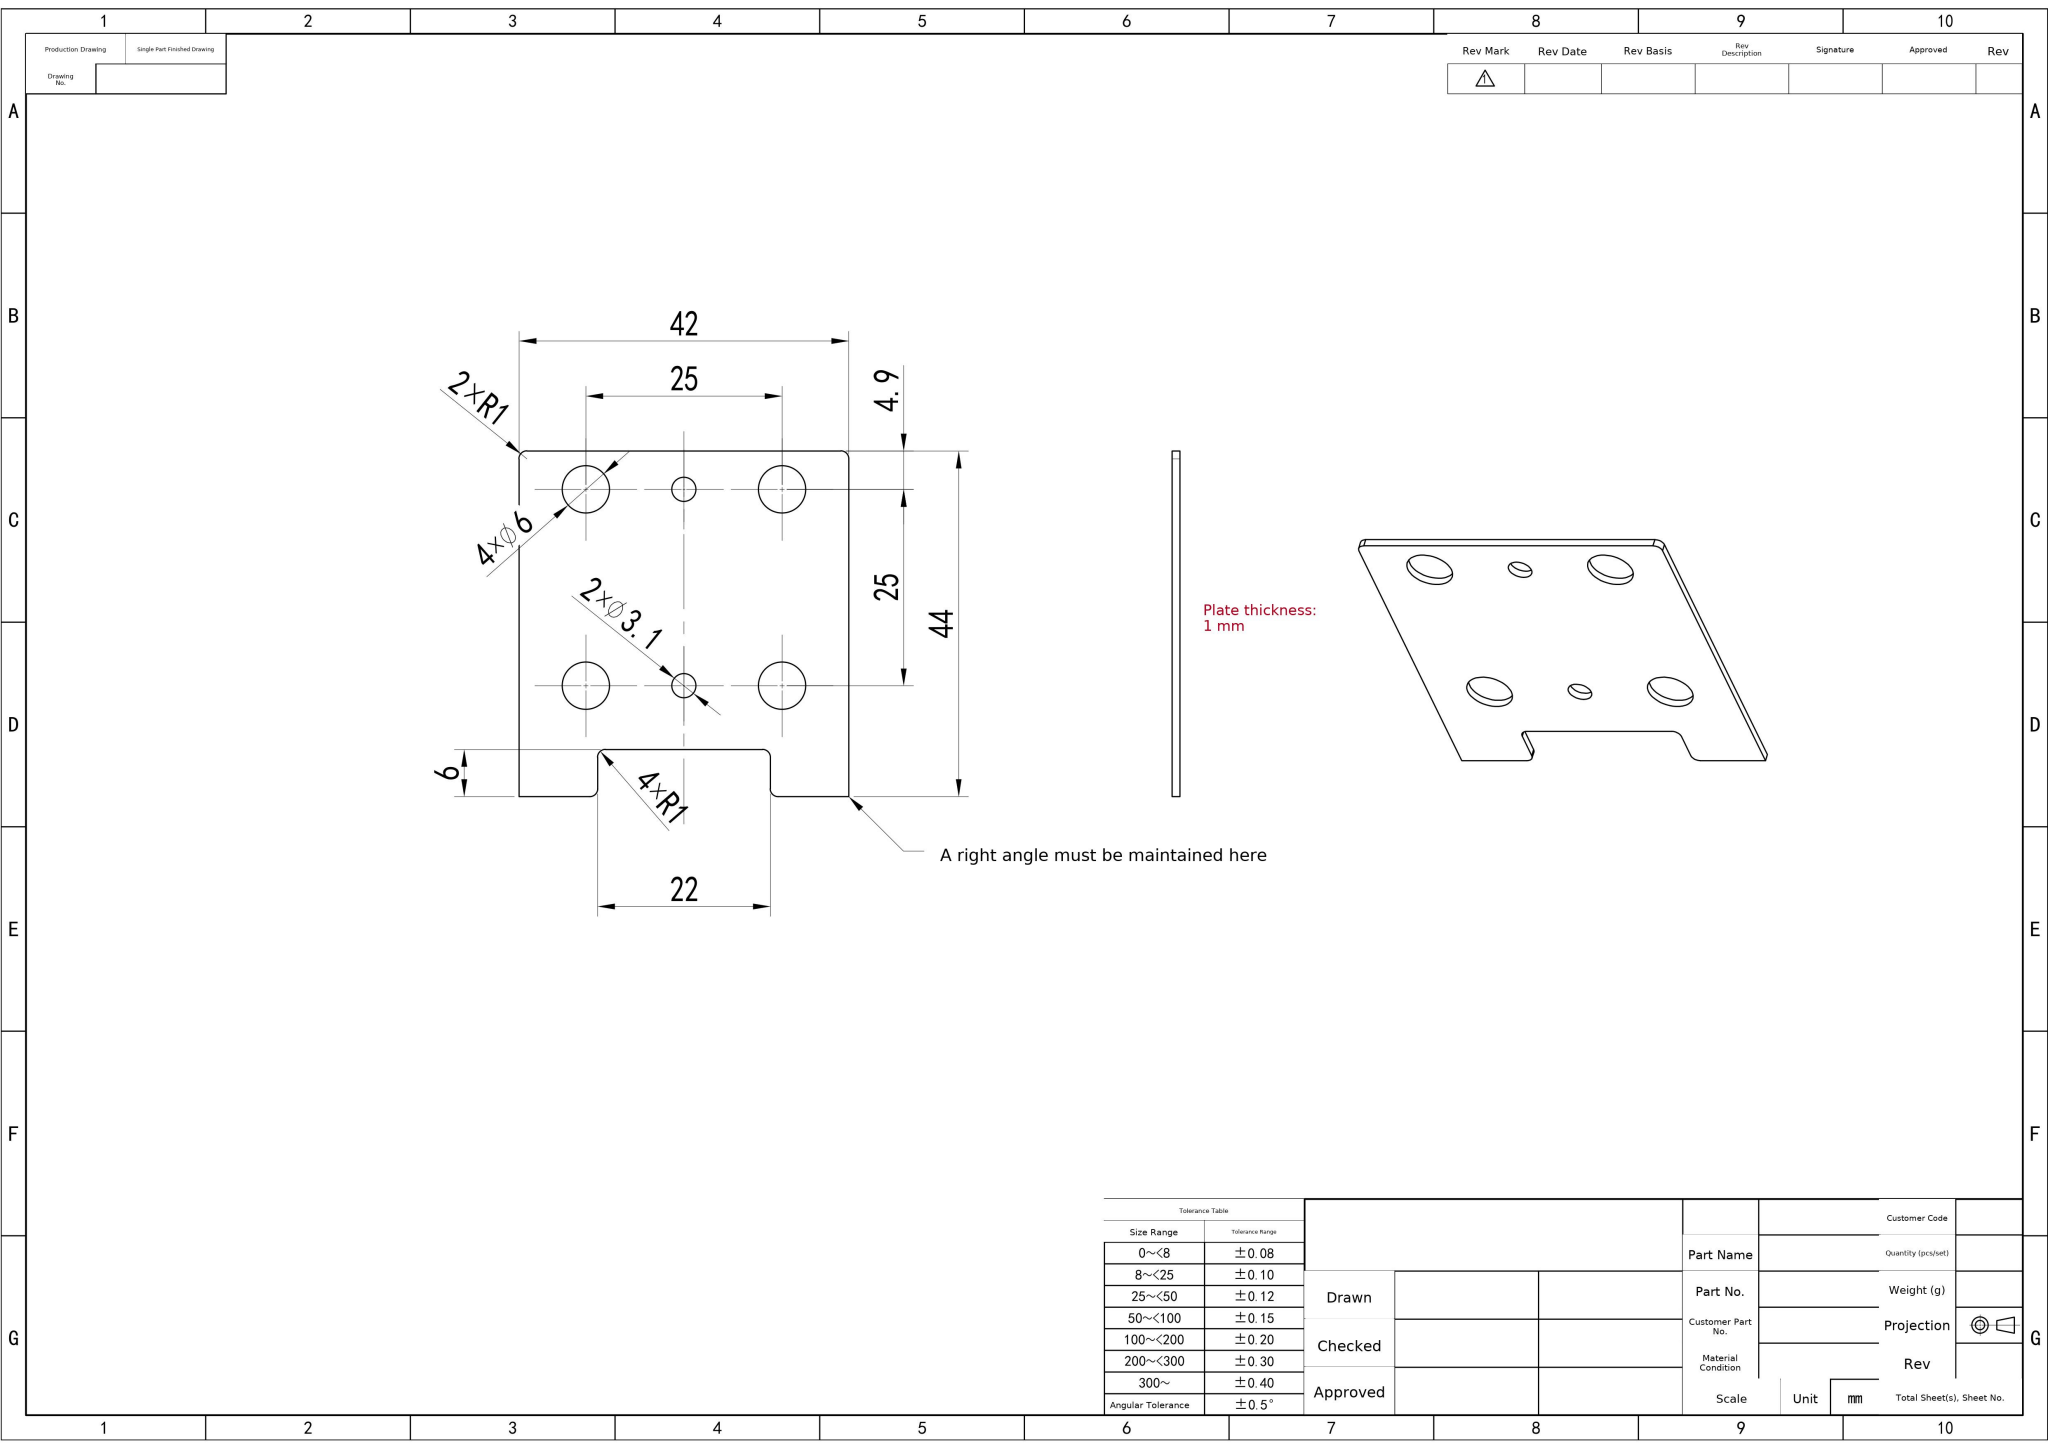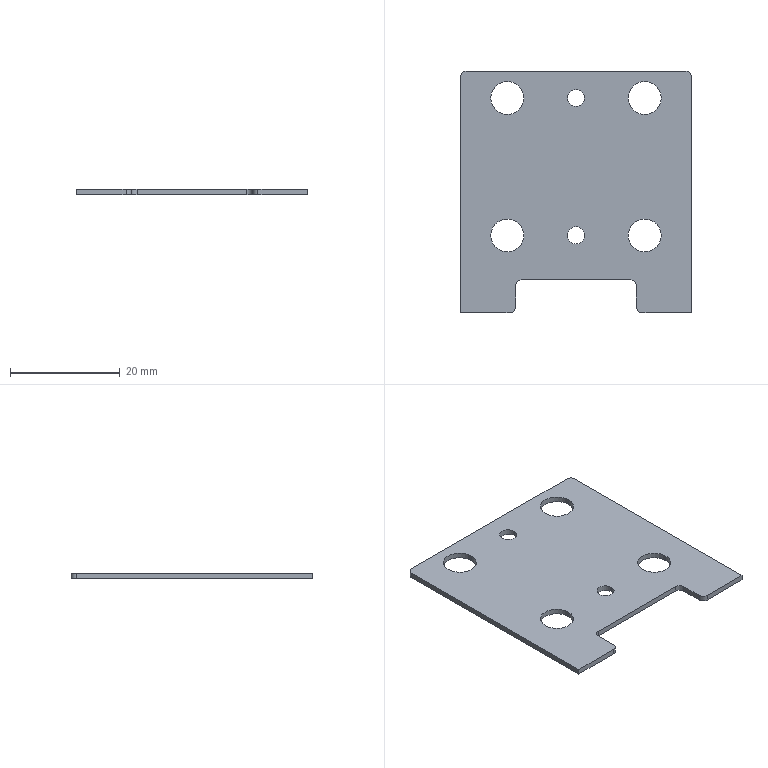Part | SolidWorks | mm | 1 solid | 28 faces | box 42 x 44 x 1 mm | volume 1587 mm3 | cylinder 18 | plane 10 | commonest cylinder face diameters 6 x8 2 x6 3.1 x4
STEP:
#1=CARTESIAN_POINT('',(15.5,0.,1.));
#2=VERTEX_POINT('',#1);
#3=CARTESIAN_POINT('',(9.5,0.,1.));
#4=VERTEX_POINT('',#3);
#5=CARTESIAN_POINT('',(12.5,0.,1.));
#6=DIRECTION('',(0.,0.,-1.));
#7=DIRECTION('',(-1.,0.,0.));
#8=AXIS2_PLACEMENT_3D('',#5,#6,#7);
#9=CIRCLE('',#8,3.);
#10=EDGE_CURVE('',#2,#4,#9,.T.);
#11=ORIENTED_EDGE('',*,*,#10,.F.);
#12=CARTESIAN_POINT('',(15.5,0.,0.));
#13=VERTEX_POINT('',#12);
#14=CARTESIAN_POINT('',(15.5,0.,1.));
#15=DIRECTION('',(0.,0.,-1.));
#16=VECTOR('',#15,1000.);
#17=LINE('',#14,#16);
#18=EDGE_CURVE('',#2,#13,#17,.T.);
#19=ORIENTED_EDGE('',*,*,#18,.T.);
#20=CARTESIAN_POINT('',(9.5,0.,0.));
#21=VERTEX_POINT('',#20);
#22=CARTESIAN_POINT('',(12.5,0.,0.));
#23=DIRECTION('',(0.,0.,1.));
#24=DIRECTION('',(-1.,0.,0.));
#25=AXIS2_PLACEMENT_3D('',#22,#23,#24);
#26=CIRCLE('',#25,3.);
#27=EDGE_CURVE('',#21,#13,#26,.T.);
#28=ORIENTED_EDGE('',*,*,#27,.F.);
#29=CARTESIAN_POINT('',(9.5,0.,1.));
#30=DIRECTION('',(0.,0.,-1.));
#31=VECTOR('',#30,1000.);
#32=LINE('',#29,#31);
#33=EDGE_CURVE('',#4,#21,#32,.T.);
#34=ORIENTED_EDGE('',*,*,#33,.F.);
#35=EDGE_LOOP('',(#11,#19,#28,#34));
#36=FACE_OUTER_BOUND('',#35,.T.);
#37=CARTESIAN_POINT('',(12.5,0.,1.));
#38=DIRECTION('',(0.,0.,-1.));
#39=DIRECTION('',(-1.,0.,0.));
#40=AXIS2_PLACEMENT_3D('',#37,#38,#39);
#41=CYLINDRICAL_SURFACE('',#40,3.);
#42=ADVANCED_FACE('',(#36),#41,.F.);
#43=CARTESIAN_POINT('',(15.5,-25.,1.));
#44=VERTEX_POINT('',#43);
#45=CARTESIAN_POINT('',(9.5,-25.,1.));
#46=VERTEX_POINT('',#45);
#47=CARTESIAN_POINT('',(12.5,-25.,1.));
#48=DIRECTION('',(0.,0.,-1.));
#49=DIRECTION('',(-1.,0.,0.));
#50=AXIS2_PLACEMENT_3D('',#47,#48,#49);
#51=CIRCLE('',#50,3.);
#52=EDGE_CURVE('',#44,#46,#51,.T.);
#53=ORIENTED_EDGE('',*,*,#52,.F.);
#54=CARTESIAN_POINT('',(15.5,-25.,0.));
#55=VERTEX_POINT('',#54);
#56=CARTESIAN_POINT('',(15.5,-25.,1.));
#57=DIRECTION('',(0.,0.,-1.));
#58=VECTOR('',#57,1000.);
#59=LINE('',#56,#58);
#60=EDGE_CURVE('',#44,#55,#59,.T.);
#61=ORIENTED_EDGE('',*,*,#60,.T.);
#62=CARTESIAN_POINT('',(9.5,-25.,0.));
#63=VERTEX_POINT('',#62);
#64=CARTESIAN_POINT('',(12.5,-25.,0.));
#65=DIRECTION('',(0.,0.,1.));
#66=DIRECTION('',(-1.,0.,0.));
#67=AXIS2_PLACEMENT_3D('',#64,#65,#66);
#68=CIRCLE('',#67,3.);
#69=EDGE_CURVE('',#63,#55,#68,.T.);
#70=ORIENTED_EDGE('',*,*,#69,.F.);
#71=CARTESIAN_POINT('',(9.5,-25.,1.));
#72=DIRECTION('',(0.,0.,-1.));
#73=VECTOR('',#72,1000.);
#74=LINE('',#71,#73);
#75=EDGE_CURVE('',#46,#63,#74,.T.);
#76=ORIENTED_EDGE('',*,*,#75,.F.);
#77=EDGE_LOOP('',(#53,#61,#70,#76));
#78=FACE_OUTER_BOUND('',#77,.T.);
#79=CARTESIAN_POINT('',(12.5,-25.,1.));
#80=DIRECTION('',(0.,0.,-1.));
#81=DIRECTION('',(-1.,0.,0.));
#82=AXIS2_PLACEMENT_3D('',#79,#80,#81);
#83=CYLINDRICAL_SURFACE('',#82,3.);
#84=ADVANCED_FACE('',(#78),#83,.F.);
#85=CARTESIAN_POINT('',(1.55,0.,1.));
#86=VERTEX_POINT('',#85);
#87=CARTESIAN_POINT('',(-1.55,0.,1.));
#88=VERTEX_POINT('',#87);
#89=CARTESIAN_POINT('',(0.,0.,1.));
#90=DIRECTION('',(0.,0.,-1.));
#91=DIRECTION('',(-1.,0.,0.));
#92=AXIS2_PLACEMENT_3D('',#89,#90,#91);
#93=CIRCLE('',#92,1.55);
#94=EDGE_CURVE('',#86,#88,#93,.T.);
#95=ORIENTED_EDGE('',*,*,#94,.F.);
#96=CARTESIAN_POINT('',(1.55,0.,0.));
#97=VERTEX_POINT('',#96);
#98=CARTESIAN_POINT('',(1.55,0.,1.));
#99=DIRECTION('',(0.,0.,-1.));
#100=VECTOR('',#99,1000.);
#101=LINE('',#98,#100);
#102=EDGE_CURVE('',#86,#97,#101,.T.);
#103=ORIENTED_EDGE('',*,*,#102,.T.);
#104=CARTESIAN_POINT('',(-1.55,0.,0.));
#105=VERTEX_POINT('',#104);
#106=CARTESIAN_POINT('',(0.,0.,0.));
#107=DIRECTION('',(0.,0.,1.));
#108=DIRECTION('',(-1.,0.,0.));
#109=AXIS2_PLACEMENT_3D('',#106,#107,#108);
#110=CIRCLE('',#109,1.55);
#111=EDGE_CURVE('',#105,#97,#110,.T.);
#112=ORIENTED_EDGE('',*,*,#111,.F.);
#113=CARTESIAN_POINT('',(-1.55,0.,1.));
#114=DIRECTION('',(0.,0.,-1.));
#115=VECTOR('',#114,1000.);
#116=LINE('',#113,#115);
#117=EDGE_CURVE('',#88,#105,#116,.T.);
#118=ORIENTED_EDGE('',*,*,#117,.F.);
#119=EDGE_LOOP('',(#95,#103,#112,#118));
#120=FACE_OUTER_BOUND('',#119,.T.);
#121=CARTESIAN_POINT('',(0.,0.,1.));
#122=DIRECTION('',(0.,0.,-1.));
#123=DIRECTION('',(-1.,0.,0.));
#124=AXIS2_PLACEMENT_3D('',#121,#122,#123);
#125=CYLINDRICAL_SURFACE('',#124,1.55);
#126=ADVANCED_FACE('',(#120),#125,.F.);
#127=CARTESIAN_POINT('',(1.55,-25.,1.));
#128=VERTEX_POINT('',#127);
#129=CARTESIAN_POINT('',(-1.55,-25.,1.));
#130=VERTEX_POINT('',#129);
#131=CARTESIAN_POINT('',(0.,-25.,1.));
#132=DIRECTION('',(0.,0.,-1.));
#133=DIRECTION('',(-1.,0.,0.));
#134=AXIS2_PLACEMENT_3D('',#131,#132,#133);
#135=CIRCLE('',#134,1.55);
#136=EDGE_CURVE('',#128,#130,#135,.T.);
#137=ORIENTED_EDGE('',*,*,#136,.F.);
#138=CARTESIAN_POINT('',(1.55,-25.,0.));
#139=VERTEX_POINT('',#138);
#140=CARTESIAN_POINT('',(1.55,-25.,1.));
#141=DIRECTION('',(0.,0.,-1.));
#142=VECTOR('',#141,1000.);
#143=LINE('',#140,#142);
#144=EDGE_CURVE('',#128,#139,#143,.T.);
#145=ORIENTED_EDGE('',*,*,#144,.T.);
#146=CARTESIAN_POINT('',(-1.55,-25.,0.));
#147=VERTEX_POINT('',#146);
#148=CARTESIAN_POINT('',(0.,-25.,0.));
#149=DIRECTION('',(0.,0.,1.));
#150=DIRECTION('',(-1.,0.,0.));
#151=AXIS2_PLACEMENT_3D('',#148,#149,#150);
#152=CIRCLE('',#151,1.55);
#153=EDGE_CURVE('',#147,#139,#152,.T.);
#154=ORIENTED_EDGE('',*,*,#153,.F.);
#155=CARTESIAN_POINT('',(-1.55,-25.,1.));
#156=DIRECTION('',(0.,0.,-1.));
#157=VECTOR('',#156,1000.);
#158=LINE('',#155,#157);
#159=EDGE_CURVE('',#130,#147,#158,.T.);
#160=ORIENTED_EDGE('',*,*,#159,.F.);
#161=EDGE_LOOP('',(#137,#145,#154,#160));
#162=FACE_OUTER_BOUND('',#161,.T.);
#163=CARTESIAN_POINT('',(0.,-25.,1.));
#164=DIRECTION('',(0.,0.,-1.));
#165=DIRECTION('',(-1.,0.,0.));
#166=AXIS2_PLACEMENT_3D('',#163,#164,#165);
#167=CYLINDRICAL_SURFACE('',#166,1.55);
#168=ADVANCED_FACE('',(#162),#167,.F.);
#169=CARTESIAN_POINT('',(-9.5,0.,1.));
#170=VERTEX_POINT('',#169);
#171=CARTESIAN_POINT('',(-15.5,0.,1.));
#172=VERTEX_POINT('',#171);
#173=CARTESIAN_POINT('',(-12.5,0.,1.));
#174=DIRECTION('',(0.,0.,-1.));
#175=DIRECTION('',(-1.,0.,0.));
#176=AXIS2_PLACEMENT_3D('',#173,#174,#175);
#177=CIRCLE('',#176,3.);
#178=EDGE_CURVE('',#170,#172,#177,.T.);
#179=ORIENTED_EDGE('',*,*,#178,.F.);
#180=CARTESIAN_POINT('',(-9.5,0.,0.));
#181=VERTEX_POINT('',#180);
#182=CARTESIAN_POINT('',(-9.5,0.,1.));
#183=DIRECTION('',(0.,0.,-1.));
#184=VECTOR('',#183,1000.);
#185=LINE('',#182,#184);
#186=EDGE_CURVE('',#170,#181,#185,.T.);
#187=ORIENTED_EDGE('',*,*,#186,.T.);
#188=CARTESIAN_POINT('',(-15.5,0.,0.));
#189=VERTEX_POINT('',#188);
#190=CARTESIAN_POINT('',(-12.5,0.,0.));
#191=DIRECTION('',(0.,0.,1.));
#192=DIRECTION('',(-1.,0.,0.));
#193=AXIS2_PLACEMENT_3D('',#190,#191,#192);
#194=CIRCLE('',#193,3.);
#195=EDGE_CURVE('',#189,#181,#194,.T.);
#196=ORIENTED_EDGE('',*,*,#195,.F.);
#197=CARTESIAN_POINT('',(-15.5,0.,1.));
#198=DIRECTION('',(0.,0.,-1.));
#199=VECTOR('',#198,1000.);
#200=LINE('',#197,#199);
#201=EDGE_CURVE('',#172,#189,#200,.T.);
#202=ORIENTED_EDGE('',*,*,#201,.F.);
#203=EDGE_LOOP('',(#179,#187,#196,#202));
#204=FACE_OUTER_BOUND('',#203,.T.);
#205=CARTESIAN_POINT('',(-12.5,0.,1.));
#206=DIRECTION('',(0.,0.,-1.));
#207=DIRECTION('',(-1.,0.,0.));
#208=AXIS2_PLACEMENT_3D('',#205,#206,#207);
#209=CYLINDRICAL_SURFACE('',#208,3.);
#210=ADVANCED_FACE('',(#204),#209,.F.);
#211=CARTESIAN_POINT('',(-9.5,-25.,1.));
#212=VERTEX_POINT('',#211);
#213=CARTESIAN_POINT('',(-15.5,-25.,1.));
#214=VERTEX_POINT('',#213);
#215=CARTESIAN_POINT('',(-12.5,-25.,1.));
#216=DIRECTION('',(0.,0.,-1.));
#217=DIRECTION('',(-1.,0.,0.));
#218=AXIS2_PLACEMENT_3D('',#215,#216,#217);
#219=CIRCLE('',#218,3.);
#220=EDGE_CURVE('',#212,#214,#219,.T.);
#221=ORIENTED_EDGE('',*,*,#220,.F.);
#222=CARTESIAN_POINT('',(-9.5,-25.,0.));
#223=VERTEX_POINT('',#222);
#224=CARTESIAN_POINT('',(-9.5,-25.,1.));
#225=DIRECTION('',(0.,0.,-1.));
#226=VECTOR('',#225,1000.);
#227=LINE('',#224,#226);
#228=EDGE_CURVE('',#212,#223,#227,.T.);
#229=ORIENTED_EDGE('',*,*,#228,.T.);
#230=CARTESIAN_POINT('',(-15.5,-25.,0.));
#231=VERTEX_POINT('',#230);
#232=CARTESIAN_POINT('',(-12.5,-25.,0.));
#233=DIRECTION('',(0.,0.,1.));
#234=DIRECTION('',(-1.,0.,0.));
#235=AXIS2_PLACEMENT_3D('',#232,#233,#234);
#236=CIRCLE('',#235,3.);
#237=EDGE_CURVE('',#231,#223,#236,.T.);
#238=ORIENTED_EDGE('',*,*,#237,.F.);
#239=CARTESIAN_POINT('',(-15.5,-25.,1.));
#240=DIRECTION('',(0.,0.,-1.));
#241=VECTOR('',#240,1000.);
#242=LINE('',#239,#241);
#243=EDGE_CURVE('',#214,#231,#242,.T.);
#244=ORIENTED_EDGE('',*,*,#243,.F.);
#245=EDGE_LOOP('',(#221,#229,#238,#244));
#246=FACE_OUTER_BOUND('',#245,.T.);
#247=CARTESIAN_POINT('',(-12.5,-25.,1.));
#248=DIRECTION('',(0.,0.,-1.));
#249=DIRECTION('',(-1.,0.,0.));
#250=AXIS2_PLACEMENT_3D('',#247,#248,#249);
#251=CYLINDRICAL_SURFACE('',#250,3.);
#252=ADVANCED_FACE('',(#246),#251,.F.);
#253=CARTESIAN_POINT('',(12.5,0.,1.));
#254=DIRECTION('',(0.,0.,-1.));
#255=DIRECTION('',(-1.,0.,0.));
#256=AXIS2_PLACEMENT_3D('',#253,#254,#255);
#257=CIRCLE('',#256,3.);
#258=EDGE_CURVE('',#4,#2,#257,.T.);
#259=ORIENTED_EDGE('',*,*,#258,.T.);
#260=ORIENTED_EDGE('',*,*,#10,.T.);
#261=EDGE_LOOP('',(#259,#260));
#262=FACE_BOUND('',#261,.T.);
#263=CARTESIAN_POINT('',(12.5,-25.,1.));
#264=DIRECTION('',(0.,0.,-1.));
#265=DIRECTION('',(-1.,0.,0.));
#266=AXIS2_PLACEMENT_3D('',#263,#264,#265);
#267=CIRCLE('',#266,3.);
#268=EDGE_CURVE('',#46,#44,#267,.T.);
#269=ORIENTED_EDGE('',*,*,#268,.T.);
#270=ORIENTED_EDGE('',*,*,#52,.T.);
#271=EDGE_LOOP('',(#269,#270));
#272=FACE_BOUND('',#271,.T.);
#273=CARTESIAN_POINT('',(0.,0.,1.));
#274=DIRECTION('',(0.,0.,-1.));
#275=DIRECTION('',(-1.,0.,0.));
#276=AXIS2_PLACEMENT_3D('',#273,#274,#275);
#277=CIRCLE('',#276,1.55);
#278=EDGE_CURVE('',#88,#86,#277,.T.);
#279=ORIENTED_EDGE('',*,*,#278,.T.);
#280=ORIENTED_EDGE('',*,*,#94,.T.);
#281=EDGE_LOOP('',(#279,#280));
#282=FACE_BOUND('',#281,.T.);
#283=CARTESIAN_POINT('',(0.,-25.,1.));
#284=DIRECTION('',(0.,0.,-1.));
#285=DIRECTION('',(-1.,0.,0.));
#286=AXIS2_PLACEMENT_3D('',#283,#284,#285);
#287=CIRCLE('',#286,1.55);
#288=EDGE_CURVE('',#130,#128,#287,.T.);
#289=ORIENTED_EDGE('',*,*,#288,.T.);
#290=ORIENTED_EDGE('',*,*,#136,.T.);
#291=EDGE_LOOP('',(#289,#290));
#292=FACE_BOUND('',#291,.T.);
#293=CARTESIAN_POINT('',(-12.5,0.,1.));
#294=DIRECTION('',(0.,0.,-1.));
#295=DIRECTION('',(-1.,0.,0.));
#296=AXIS2_PLACEMENT_3D('',#293,#294,#295);
#297=CIRCLE('',#296,3.);
#298=EDGE_CURVE('',#172,#170,#297,.T.);
#299=ORIENTED_EDGE('',*,*,#298,.T.);
#300=ORIENTED_EDGE('',*,*,#178,.T.);
#301=EDGE_LOOP('',(#299,#300));
#302=FACE_BOUND('',#301,.T.);
#303=CARTESIAN_POINT('',(-12.5,-25.,1.));
#304=DIRECTION('',(0.,0.,-1.));
#305=DIRECTION('',(-1.,0.,0.));
#306=AXIS2_PLACEMENT_3D('',#303,#304,#305);
#307=CIRCLE('',#306,3.);
#308=EDGE_CURVE('',#214,#212,#307,.T.);
#309=ORIENTED_EDGE('',*,*,#308,.T.);
#310=ORIENTED_EDGE('',*,*,#220,.T.);
#311=EDGE_LOOP('',(#309,#310));
#312=FACE_BOUND('',#311,.T.);
#313=CARTESIAN_POINT('',(20.,4.9,1.));
#314=VERTEX_POINT('',#313);
#315=CARTESIAN_POINT('',(-20.,4.9,1.));
#316=VERTEX_POINT('',#315);
#317=CARTESIAN_POINT('',(-12.,4.9,1.));
#318=DIRECTION('',(-1.,0.,0.));
#319=VECTOR('',#318,1000.);
#320=LINE('',#317,#319);
#321=EDGE_CURVE('',#314,#316,#320,.T.);
#322=ORIENTED_EDGE('',*,*,#321,.T.);
#323=CARTESIAN_POINT('',(-21.,3.9,1.));
#324=VERTEX_POINT('',#323);
#325=CARTESIAN_POINT('',(-20.,3.9,1.));
#326=DIRECTION('',(0.,0.,1.));
#327=DIRECTION('',(-1.,0.,0.));
#328=AXIS2_PLACEMENT_3D('',#325,#326,#327);
#329=CIRCLE('',#328,1.);
#330=EDGE_CURVE('',#316,#324,#329,.T.);
#331=ORIENTED_EDGE('',*,*,#330,.T.);
#332=CARTESIAN_POINT('',(-21.,-39.1,1.));
#333=VERTEX_POINT('',#332);
#334=CARTESIAN_POINT('',(-21.,-38.1,1.));
#335=DIRECTION('',(0.,-1.,0.));
#336=VECTOR('',#335,1000.);
#337=LINE('',#334,#336);
#338=EDGE_CURVE('',#324,#333,#337,.T.);
#339=ORIENTED_EDGE('',*,*,#338,.T.);
#340=CARTESIAN_POINT('',(-12.,-39.1,1.));
#341=VERTEX_POINT('',#340);
#342=CARTESIAN_POINT('',(-12.,-39.1,1.));
#343=DIRECTION('',(1.,0.,0.));
#344=VECTOR('',#343,1000.);
#345=LINE('',#342,#344);
#346=EDGE_CURVE('',#333,#341,#345,.T.);
#347=ORIENTED_EDGE('',*,*,#346,.T.);
#348=CARTESIAN_POINT('',(-11.,-38.1,1.));
#349=VERTEX_POINT('',#348);
#350=CARTESIAN_POINT('',(-12.,-38.1,1.));
#351=DIRECTION('',(0.,0.,1.));
#352=DIRECTION('',(-1.,0.,0.));
#353=AXIS2_PLACEMENT_3D('',#350,#351,#352);
#354=CIRCLE('',#353,1.);
#355=EDGE_CURVE('',#341,#349,#354,.T.);
#356=ORIENTED_EDGE('',*,*,#355,.T.);
#357=CARTESIAN_POINT('',(-11.,-34.1,1.));
#358=VERTEX_POINT('',#357);
#359=CARTESIAN_POINT('',(-11.,-38.1,1.));
#360=DIRECTION('',(0.,1.,0.));
#361=VECTOR('',#360,1000.);
#362=LINE('',#359,#361);
#363=EDGE_CURVE('',#349,#358,#362,.T.);
#364=ORIENTED_EDGE('',*,*,#363,.T.);
#365=CARTESIAN_POINT('',(-10.,-33.1,1.));
#366=VERTEX_POINT('',#365);
#367=CARTESIAN_POINT('',(-10.,-34.1,1.));
#368=DIRECTION('',(0.,0.,-1.));
#369=DIRECTION('',(-1.,0.,0.));
#370=AXIS2_PLACEMENT_3D('',#367,#368,#369);
#371=CIRCLE('',#370,1.);
#372=EDGE_CURVE('',#358,#366,#371,.T.);
#373=ORIENTED_EDGE('',*,*,#372,.T.);
#374=CARTESIAN_POINT('',(10.,-33.1,1.));
#375=VERTEX_POINT('',#374);
#376=CARTESIAN_POINT('',(-12.,-33.1,1.));
#377=DIRECTION('',(1.,0.,0.));
#378=VECTOR('',#377,1000.);
#379=LINE('',#376,#378);
#380=EDGE_CURVE('',#366,#375,#379,.T.);
#381=ORIENTED_EDGE('',*,*,#380,.T.);
#382=CARTESIAN_POINT('',(11.,-34.1,1.));
#383=VERTEX_POINT('',#382);
#384=CARTESIAN_POINT('',(10.,-34.1,1.));
#385=DIRECTION('',(0.,0.,-1.));
#386=DIRECTION('',(-1.,0.,0.));
#387=AXIS2_PLACEMENT_3D('',#384,#385,#386);
#388=CIRCLE('',#387,1.);
#389=EDGE_CURVE('',#375,#383,#388,.T.);
#390=ORIENTED_EDGE('',*,*,#389,.T.);
#391=CARTESIAN_POINT('',(11.,-38.1,1.));
#392=VERTEX_POINT('',#391);
#393=CARTESIAN_POINT('',(11.,-38.1,1.));
#394=DIRECTION('',(0.,-1.,0.));
#395=VECTOR('',#394,1000.);
#396=LINE('',#393,#395);
#397=EDGE_CURVE('',#383,#392,#396,.T.);
#398=ORIENTED_EDGE('',*,*,#397,.T.);
#399=CARTESIAN_POINT('',(12.,-39.1,1.));
#400=VERTEX_POINT('',#399);
#401=CARTESIAN_POINT('',(12.,-38.1,1.));
#402=DIRECTION('',(0.,0.,1.));
#403=DIRECTION('',(-1.,0.,0.));
#404=AXIS2_PLACEMENT_3D('',#401,#402,#403);
#405=CIRCLE('',#404,1.);
#406=EDGE_CURVE('',#392,#400,#405,.T.);
#407=ORIENTED_EDGE('',*,*,#406,.T.);
#408=CARTESIAN_POINT('',(21.,-39.1,1.));
#409=VERTEX_POINT('',#408);
#410=CARTESIAN_POINT('',(-12.,-39.1,1.));
#411=DIRECTION('',(1.,0.,0.));
#412=VECTOR('',#411,1000.);
#413=LINE('',#410,#412);
#414=EDGE_CURVE('',#400,#409,#413,.T.);
#415=ORIENTED_EDGE('',*,*,#414,.T.);
#416=CARTESIAN_POINT('',(21.,3.9,1.));
#417=VERTEX_POINT('',#416);
#418=CARTESIAN_POINT('',(21.,-38.1,1.));
#419=DIRECTION('',(0.,1.,0.));
#420=VECTOR('',#419,1000.);
#421=LINE('',#418,#420);
#422=EDGE_CURVE('',#409,#417,#421,.T.);
#423=ORIENTED_EDGE('',*,*,#422,.T.);
#424=CARTESIAN_POINT('',(20.,3.9,1.));
#425=DIRECTION('',(0.,0.,1.));
#426=DIRECTION('',(-1.,0.,0.));
#427=AXIS2_PLACEMENT_3D('',#424,#425,#426);
#428=CIRCLE('',#427,1.);
#429=EDGE_CURVE('',#417,#314,#428,.T.);
#430=ORIENTED_EDGE('',*,*,#429,.T.);
#431=EDGE_LOOP('',(#322,#331,#339,#347,#356,#364,#373,#381,#390,#398,#407,#415,#423,#430));
#432=FACE_OUTER_BOUND('',#431,.T.);
#433=CARTESIAN_POINT('',(-12.,-38.1,1.));
#434=DIRECTION('',(0.,0.,1.));
#435=DIRECTION('',(1.,0.,0.));
#436=AXIS2_PLACEMENT_3D('',#433,#434,#435);
#437=PLANE('',#436);
#438=ADVANCED_FACE('',(#262,#272,#282,#292,#302,#312,#432),#437,.T.);
#439=ORIENTED_EDGE('',*,*,#18,.F.);
#440=ORIENTED_EDGE('',*,*,#258,.F.);
#441=ORIENTED_EDGE('',*,*,#33,.T.);
#442=CARTESIAN_POINT('',(12.5,0.,0.));
#443=DIRECTION('',(0.,0.,1.));
#444=DIRECTION('',(-1.,0.,0.));
#445=AXIS2_PLACEMENT_3D('',#442,#443,#444);
#446=CIRCLE('',#445,3.);
#447=EDGE_CURVE('',#13,#21,#446,.T.);
#448=ORIENTED_EDGE('',*,*,#447,.F.);
#449=EDGE_LOOP('',(#439,#440,#441,#448));
#450=FACE_OUTER_BOUND('',#449,.T.);
#451=CARTESIAN_POINT('',(12.5,0.,1.));
#452=DIRECTION('',(0.,0.,-1.));
#453=DIRECTION('',(-1.,0.,0.));
#454=AXIS2_PLACEMENT_3D('',#451,#452,#453);
#455=CYLINDRICAL_SURFACE('',#454,3.);
#456=ADVANCED_FACE('',(#450),#455,.F.);
#457=ORIENTED_EDGE('',*,*,#60,.F.);
#458=ORIENTED_EDGE('',*,*,#268,.F.);
#459=ORIENTED_EDGE('',*,*,#75,.T.);
#460=CARTESIAN_POINT('',(12.5,-25.,0.));
#461=DIRECTION('',(0.,0.,1.));
#462=DIRECTION('',(-1.,0.,0.));
#463=AXIS2_PLACEMENT_3D('',#460,#461,#462);
#464=CIRCLE('',#463,3.);
#465=EDGE_CURVE('',#55,#63,#464,.T.);
#466=ORIENTED_EDGE('',*,*,#465,.F.);
#467=EDGE_LOOP('',(#457,#458,#459,#466));
#468=FACE_OUTER_BOUND('',#467,.T.);
#469=CARTESIAN_POINT('',(12.5,-25.,1.));
#470=DIRECTION('',(0.,0.,-1.));
#471=DIRECTION('',(-1.,0.,0.));
#472=AXIS2_PLACEMENT_3D('',#469,#470,#471);
#473=CYLINDRICAL_SURFACE('',#472,3.);
#474=ADVANCED_FACE('',(#468),#473,.F.);
#475=ORIENTED_EDGE('',*,*,#102,.F.);
#476=ORIENTED_EDGE('',*,*,#278,.F.);
#477=ORIENTED_EDGE('',*,*,#117,.T.);
#478=CARTESIAN_POINT('',(0.,0.,0.));
#479=DIRECTION('',(0.,0.,1.));
#480=DIRECTION('',(-1.,0.,0.));
#481=AXIS2_PLACEMENT_3D('',#478,#479,#480);
#482=CIRCLE('',#481,1.55);
#483=EDGE_CURVE('',#97,#105,#482,.T.);
#484=ORIENTED_EDGE('',*,*,#483,.F.);
#485=EDGE_LOOP('',(#475,#476,#477,#484));
#486=FACE_OUTER_BOUND('',#485,.T.);
#487=CARTESIAN_POINT('',(0.,0.,1.));
#488=DIRECTION('',(0.,0.,-1.));
#489=DIRECTION('',(-1.,0.,0.));
#490=AXIS2_PLACEMENT_3D('',#487,#488,#489);
#491=CYLINDRICAL_SURFACE('',#490,1.55);
#492=ADVANCED_FACE('',(#486),#491,.F.);
#493=ORIENTED_EDGE('',*,*,#144,.F.);
#494=ORIENTED_EDGE('',*,*,#288,.F.);
#495=ORIENTED_EDGE('',*,*,#159,.T.);
#496=CARTESIAN_POINT('',(0.,-25.,0.));
#497=DIRECTION('',(0.,0.,1.));
#498=DIRECTION('',(-1.,0.,0.));
#499=AXIS2_PLACEMENT_3D('',#496,#497,#498);
#500=CIRCLE('',#499,1.55);
#501=EDGE_CURVE('',#139,#147,#500,.T.);
#502=ORIENTED_EDGE('',*,*,#501,.F.);
#503=EDGE_LOOP('',(#493,#494,#495,#502));
#504=FACE_OUTER_BOUND('',#503,.T.);
#505=CARTESIAN_POINT('',(0.,-25.,1.));
#506=DIRECTION('',(0.,0.,-1.));
#507=DIRECTION('',(-1.,0.,0.));
#508=AXIS2_PLACEMENT_3D('',#505,#506,#507);
#509=CYLINDRICAL_SURFACE('',#508,1.55);
#510=ADVANCED_FACE('',(#504),#509,.F.);
#511=ORIENTED_EDGE('',*,*,#186,.F.);
#512=ORIENTED_EDGE('',*,*,#298,.F.);
#513=ORIENTED_EDGE('',*,*,#201,.T.);
#514=CARTESIAN_POINT('',(-12.5,0.,0.));
#515=DIRECTION('',(0.,0.,1.));
#516=DIRECTION('',(-1.,0.,0.));
#517=AXIS2_PLACEMENT_3D('',#514,#515,#516);
#518=CIRCLE('',#517,3.);
#519=EDGE_CURVE('',#181,#189,#518,.T.);
#520=ORIENTED_EDGE('',*,*,#519,.F.);
#521=EDGE_LOOP('',(#511,#512,#513,#520));
#522=FACE_OUTER_BOUND('',#521,.T.);
#523=CARTESIAN_POINT('',(-12.5,0.,1.));
#524=DIRECTION('',(0.,0.,-1.));
#525=DIRECTION('',(-1.,0.,0.));
#526=AXIS2_PLACEMENT_3D('',#523,#524,#525);
#527=CYLINDRICAL_SURFACE('',#526,3.);
#528=ADVANCED_FACE('',(#522),#527,.F.);
#529=ORIENTED_EDGE('',*,*,#228,.F.);
#530=ORIENTED_EDGE('',*,*,#308,.F.);
#531=ORIENTED_EDGE('',*,*,#243,.T.);
#532=CARTESIAN_POINT('',(-12.5,-25.,0.));
#533=DIRECTION('',(0.,0.,1.));
#534=DIRECTION('',(-1.,0.,0.));
#535=AXIS2_PLACEMENT_3D('',#532,#533,#534);
#536=CIRCLE('',#535,3.);
#537=EDGE_CURVE('',#223,#231,#536,.T.);
#538=ORIENTED_EDGE('',*,*,#537,.F.);
#539=EDGE_LOOP('',(#529,#530,#531,#538));
#540=FACE_OUTER_BOUND('',#539,.T.);
#541=CARTESIAN_POINT('',(-12.5,-25.,1.));
#542=DIRECTION('',(0.,0.,-1.));
#543=DIRECTION('',(-1.,0.,0.));
#544=AXIS2_PLACEMENT_3D('',#541,#542,#543);
#545=CYLINDRICAL_SURFACE('',#544,3.);
#546=ADVANCED_FACE('',(#540),#545,.F.);
#547=ORIENTED_EDGE('',*,*,#330,.F.);
#548=CARTESIAN_POINT('',(-20.,4.9,0.));
#549=VERTEX_POINT('',#548);
#550=CARTESIAN_POINT('',(-20.,4.9,1.));
#551=DIRECTION('',(0.,0.,-1.));
#552=VECTOR('',#551,1000.);
#553=LINE('',#550,#552);
#554=EDGE_CURVE('',#316,#549,#553,.T.);
#555=ORIENTED_EDGE('',*,*,#554,.T.);
#556=CARTESIAN_POINT('',(-21.,3.9,0.));
#557=VERTEX_POINT('',#556);
#558=CARTESIAN_POINT('',(-20.,3.9,0.));
#559=DIRECTION('',(0.,0.,1.));
#560=DIRECTION('',(-1.,0.,0.));
#561=AXIS2_PLACEMENT_3D('',#558,#559,#560);
#562=CIRCLE('',#561,1.);
#563=EDGE_CURVE('',#549,#557,#562,.T.);
#564=ORIENTED_EDGE('',*,*,#563,.T.);
#565=CARTESIAN_POINT('',(-21.,3.9,1.));
#566=DIRECTION('',(0.,0.,1.));
#567=VECTOR('',#566,1000.);
#568=LINE('',#565,#567);
#569=EDGE_CURVE('',#557,#324,#568,.T.);
#570=ORIENTED_EDGE('',*,*,#569,.T.);
#571=EDGE_LOOP('',(#547,#555,#564,#570));
#572=FACE_OUTER_BOUND('',#571,.T.);
#573=CARTESIAN_POINT('',(-20.,3.9,1.));
#574=DIRECTION('',(0.,0.,-1.));
#575=DIRECTION('',(-1.,0.,0.));
#576=AXIS2_PLACEMENT_3D('',#573,#574,#575);
#577=CYLINDRICAL_SURFACE('',#576,1.);
#578=ADVANCED_FACE('',(#572),#577,.T.);
#579=ORIENTED_EDGE('',*,*,#554,.F.);
#580=ORIENTED_EDGE('',*,*,#321,.F.);
#581=CARTESIAN_POINT('',(20.,4.9,0.));
#582=VERTEX_POINT('',#581);
#583=CARTESIAN_POINT('',(20.,4.9,1.));
#584=DIRECTION('',(0.,0.,1.));
#585=VECTOR('',#584,1000.);
#586=LINE('',#583,#585);
#587=EDGE_CURVE('',#582,#314,#586,.T.);
#588=ORIENTED_EDGE('',*,*,#587,.F.);
#589=CARTESIAN_POINT('',(20.,4.9,0.));
#590=DIRECTION('',(1.,0.,0.));
#591=VECTOR('',#590,1000.);
#592=LINE('',#589,#591);
#593=EDGE_CURVE('',#549,#582,#592,.T.);
#594=ORIENTED_EDGE('',*,*,#593,.F.);
#595=EDGE_LOOP('',(#579,#580,#588,#594));
#596=FACE_OUTER_BOUND('',#595,.T.);
#597=CARTESIAN_POINT('',(20.,4.9,1.));
#598=DIRECTION('',(0.,-1.,0.));
#599=DIRECTION('',(0.,0.,-1.));
#600=AXIS2_PLACEMENT_3D('',#597,#598,#599);
#601=PLANE('',#600);
#602=ADVANCED_FACE('',(#596),#601,.F.);
#603=ORIENTED_EDGE('',*,*,#429,.F.);
#604=CARTESIAN_POINT('',(21.,3.9,0.));
#605=VERTEX_POINT('',#604);
#606=CARTESIAN_POINT('',(21.,3.9,1.));
#607=DIRECTION('',(0.,0.,-1.));
#608=VECTOR('',#607,1000.);
#609=LINE('',#606,#608);
#610=EDGE_CURVE('',#417,#605,#609,.T.);
#611=ORIENTED_EDGE('',*,*,#610,.T.);
#612=CARTESIAN_POINT('',(20.,3.9,0.));
#613=DIRECTION('',(0.,0.,1.));
#614=DIRECTION('',(-1.,0.,0.));
#615=AXIS2_PLACEMENT_3D('',#612,#613,#614);
#616=CIRCLE('',#615,1.);
#617=EDGE_CURVE('',#605,#582,#616,.T.);
#618=ORIENTED_EDGE('',*,*,#617,.T.);
#619=ORIENTED_EDGE('',*,*,#587,.T.);
#620=EDGE_LOOP('',(#603,#611,#618,#619));
#621=FACE_OUTER_BOUND('',#620,.T.);
#622=CARTESIAN_POINT('',(20.,3.9,1.));
#623=DIRECTION('',(0.,0.,-1.));
#624=DIRECTION('',(-1.,0.,0.));
#625=AXIS2_PLACEMENT_3D('',#622,#623,#624);
#626=CYLINDRICAL_SURFACE('',#625,1.);
#627=ADVANCED_FACE('',(#621),#626,.T.);
#628=ORIENTED_EDGE('',*,*,#610,.F.);
#629=ORIENTED_EDGE('',*,*,#422,.F.);
#630=CARTESIAN_POINT('',(21.,-39.1,0.));
#631=VERTEX_POINT('',#630);
#632=CARTESIAN_POINT('',(21.,-39.1,1.));
#633=DIRECTION('',(0.,0.,1.));
#634=VECTOR('',#633,1000.);
#635=LINE('',#632,#634);
#636=EDGE_CURVE('',#631,#409,#635,.T.);
#637=ORIENTED_EDGE('',*,*,#636,.F.);
#638=CARTESIAN_POINT('',(21.,-39.1,0.));
#639=DIRECTION('',(0.,-1.,0.));
#640=VECTOR('',#639,1000.);
#641=LINE('',#638,#640);
#642=EDGE_CURVE('',#605,#631,#641,.T.);
#643=ORIENTED_EDGE('',*,*,#642,.F.);
#644=EDGE_LOOP('',(#628,#629,#637,#643));
#645=FACE_OUTER_BOUND('',#644,.T.);
#646=CARTESIAN_POINT('',(21.,-39.1,1.));
#647=DIRECTION('',(-1.,0.,0.));
#648=DIRECTION('',(0.,0.,1.));
#649=AXIS2_PLACEMENT_3D('',#646,#647,#648);
#650=PLANE('',#649);
#651=ADVANCED_FACE('',(#645),#650,.F.);
#652=ORIENTED_EDGE('',*,*,#636,.T.);
#653=ORIENTED_EDGE('',*,*,#414,.F.);
#654=CARTESIAN_POINT('',(12.,-39.1,0.));
#655=VERTEX_POINT('',#654);
#656=CARTESIAN_POINT('',(12.,-39.1,1.));
#657=DIRECTION('',(0.,0.,1.));
#658=VECTOR('',#657,1000.);
#659=LINE('',#656,#658);
#660=EDGE_CURVE('',#655,#400,#659,.T.);
#661=ORIENTED_EDGE('',*,*,#660,.F.);
#662=CARTESIAN_POINT('',(12.,-39.1,0.));
#663=DIRECTION('',(-1.,0.,0.));
#664=VECTOR('',#663,1000.);
#665=LINE('',#662,#664);
#666=EDGE_CURVE('',#631,#655,#665,.T.);
#667=ORIENTED_EDGE('',*,*,#666,.F.);
#668=EDGE_LOOP('',(#652,#653,#661,#667));
#669=FACE_OUTER_BOUND('',#668,.T.);
#670=CARTESIAN_POINT('',(12.,-39.1,1.));
#671=DIRECTION('',(0.,1.,0.));
#672=DIRECTION('',(0.,0.,1.));
#673=AXIS2_PLACEMENT_3D('',#670,#671,#672);
#674=PLANE('',#673);
#675=ADVANCED_FACE('',(#669),#674,.F.);
#676=ORIENTED_EDGE('',*,*,#406,.F.);
#677=CARTESIAN_POINT('',(11.,-38.1,0.));
#678=VERTEX_POINT('',#677);
#679=CARTESIAN_POINT('',(11.,-38.1,1.));
#680=DIRECTION('',(0.,0.,-1.));
#681=VECTOR('',#680,1000.);
#682=LINE('',#679,#681);
#683=EDGE_CURVE('',#392,#678,#682,.T.);
#684=ORIENTED_EDGE('',*,*,#683,.T.);
#685=CARTESIAN_POINT('',(12.,-38.1,0.));
#686=DIRECTION('',(0.,0.,1.));
#687=DIRECTION('',(-1.,0.,0.));
#688=AXIS2_PLACEMENT_3D('',#685,#686,#687);
#689=CIRCLE('',#688,1.);
#690=EDGE_CURVE('',#678,#655,#689,.T.);
#691=ORIENTED_EDGE('',*,*,#690,.T.);
#692=ORIENTED_EDGE('',*,*,#660,.T.);
#693=EDGE_LOOP('',(#676,#684,#691,#692));
#694=FACE_OUTER_BOUND('',#693,.T.);
#695=CARTESIAN_POINT('',(12.,-38.1,1.));
#696=DIRECTION('',(0.,0.,-1.));
#697=DIRECTION('',(-1.,0.,0.));
#698=AXIS2_PLACEMENT_3D('',#695,#696,#697);
#699=CYLINDRICAL_SURFACE('',#698,1.);
#700=ADVANCED_FACE('',(#694),#699,.T.);
#701=ORIENTED_EDGE('',*,*,#683,.F.);
#702=ORIENTED_EDGE('',*,*,#397,.F.);
#703=CARTESIAN_POINT('',(11.,-34.1,0.));
#704=VERTEX_POINT('',#703);
#705=CARTESIAN_POINT('',(11.,-34.1,1.));
#706=DIRECTION('',(0.,0.,1.));
#707=VECTOR('',#706,1000.);
#708=LINE('',#705,#707);
#709=EDGE_CURVE('',#704,#383,#708,.T.);
#710=ORIENTED_EDGE('',*,*,#709,.F.);
#711=CARTESIAN_POINT('',(11.,-34.1,0.));
#712=DIRECTION('',(0.,1.,0.));
#713=VECTOR('',#712,1000.);
#714=LINE('',#711,#713);
#715=EDGE_CURVE('',#678,#704,#714,.T.);
#716=ORIENTED_EDGE('',*,*,#715,.F.);
#717=EDGE_LOOP('',(#701,#702,#710,#716));
#718=FACE_OUTER_BOUND('',#717,.T.);
#719=CARTESIAN_POINT('',(11.,-34.1,1.));
#720=DIRECTION('',(1.,0.,0.));
#721=DIRECTION('',(0.,0.,-1.));
#722=AXIS2_PLACEMENT_3D('',#719,#720,#721);
#723=PLANE('',#722);
#724=ADVANCED_FACE('',(#718),#723,.F.);
#725=ORIENTED_EDGE('',*,*,#709,.T.);
#726=ORIENTED_EDGE('',*,*,#389,.F.);
#727=CARTESIAN_POINT('',(10.,-33.1,0.));
#728=VERTEX_POINT('',#727);
#729=CARTESIAN_POINT('',(10.,-33.1,1.));
#730=DIRECTION('',(0.,0.,1.));
#731=VECTOR('',#730,1000.);
#732=LINE('',#729,#731);
#733=EDGE_CURVE('',#728,#375,#732,.T.);
#734=ORIENTED_EDGE('',*,*,#733,.F.);
#735=CARTESIAN_POINT('',(10.,-34.1,0.));
#736=DIRECTION('',(0.,0.,1.));
#737=DIRECTION('',(-1.,0.,0.));
#738=AXIS2_PLACEMENT_3D('',#735,#736,#737);
#739=CIRCLE('',#738,1.);
#740=EDGE_CURVE('',#704,#728,#739,.T.);
#741=ORIENTED_EDGE('',*,*,#740,.F.);
#742=EDGE_LOOP('',(#725,#726,#734,#741));
#743=FACE_OUTER_BOUND('',#742,.T.);
#744=CARTESIAN_POINT('',(10.,-34.1,1.));
#745=DIRECTION('',(0.,0.,-1.));
#746=DIRECTION('',(-1.,0.,0.));
#747=AXIS2_PLACEMENT_3D('',#744,#745,#746);
#748=CYLINDRICAL_SURFACE('',#747,1.);
#749=ADVANCED_FACE('',(#743),#748,.F.);
#750=ORIENTED_EDGE('',*,*,#733,.T.);
#751=ORIENTED_EDGE('',*,*,#380,.F.);
#752=CARTESIAN_POINT('',(-10.,-33.1,0.));
#753=VERTEX_POINT('',#752);
#754=CARTESIAN_POINT('',(-10.,-33.1,1.));
#755=DIRECTION('',(0.,0.,1.));
#756=VECTOR('',#755,1000.);
#757=LINE('',#754,#756);
#758=EDGE_CURVE('',#753,#366,#757,.T.);
#759=ORIENTED_EDGE('',*,*,#758,.F.);
#760=CARTESIAN_POINT('',(-10.,-33.1,0.));
#761=DIRECTION('',(-1.,0.,0.));
#762=VECTOR('',#761,1000.);
#763=LINE('',#760,#762);
#764=EDGE_CURVE('',#728,#753,#763,.T.);
#765=ORIENTED_EDGE('',*,*,#764,.F.);
#766=EDGE_LOOP('',(#750,#751,#759,#765));
#767=FACE_OUTER_BOUND('',#766,.T.);
#768=CARTESIAN_POINT('',(-10.,-33.1,1.));
#769=DIRECTION('',(0.,1.,0.));
#770=DIRECTION('',(0.,0.,1.));
#771=AXIS2_PLACEMENT_3D('',#768,#769,#770);
#772=PLANE('',#771);
#773=ADVANCED_FACE('',(#767),#772,.F.);
#774=ORIENTED_EDGE('',*,*,#758,.T.);
#775=ORIENTED_EDGE('',*,*,#372,.F.);
#776=CARTESIAN_POINT('',(-11.,-34.1,0.));
#777=VERTEX_POINT('',#776);
#778=CARTESIAN_POINT('',(-11.,-34.1,1.));
#779=DIRECTION('',(0.,0.,1.));
#780=VECTOR('',#779,1000.);
#781=LINE('',#778,#780);
#782=EDGE_CURVE('',#777,#358,#781,.T.);
#783=ORIENTED_EDGE('',*,*,#782,.F.);
#784=CARTESIAN_POINT('',(-10.,-34.1,0.));
#785=DIRECTION('',(0.,0.,1.));
#786=DIRECTION('',(-1.,0.,0.));
#787=AXIS2_PLACEMENT_3D('',#784,#785,#786);
#788=CIRCLE('',#787,1.);
#789=EDGE_CURVE('',#753,#777,#788,.T.);
#790=ORIENTED_EDGE('',*,*,#789,.F.);
#791=EDGE_LOOP('',(#774,#775,#783,#790));
#792=FACE_OUTER_BOUND('',#791,.T.);
#793=CARTESIAN_POINT('',(-10.,-34.1,1.));
#794=DIRECTION('',(0.,0.,-1.));
#795=DIRECTION('',(-1.,0.,0.));
#796=AXIS2_PLACEMENT_3D('',#793,#794,#795);
#797=CYLINDRICAL_SURFACE('',#796,1.);
#798=ADVANCED_FACE('',(#792),#797,.F.);
#799=ORIENTED_EDGE('',*,*,#782,.T.);
#800=ORIENTED_EDGE('',*,*,#363,.F.);
#801=CARTESIAN_POINT('',(-11.,-38.1,0.));
#802=VERTEX_POINT('',#801);
#803=CARTESIAN_POINT('',(-11.,-38.1,1.));
#804=DIRECTION('',(0.,0.,1.));
#805=VECTOR('',#804,1000.);
#806=LINE('',#803,#805);
#807=EDGE_CURVE('',#802,#349,#806,.T.);
#808=ORIENTED_EDGE('',*,*,#807,.F.);
#809=CARTESIAN_POINT('',(-11.,-38.1,0.));
#810=DIRECTION('',(0.,-1.,0.));
#811=VECTOR('',#810,1000.);
#812=LINE('',#809,#811);
#813=EDGE_CURVE('',#777,#802,#812,.T.);
#814=ORIENTED_EDGE('',*,*,#813,.F.);
#815=EDGE_LOOP('',(#799,#800,#808,#814));
#816=FACE_OUTER_BOUND('',#815,.T.);
#817=CARTESIAN_POINT('',(-11.,-38.1,1.));
#818=DIRECTION('',(-1.,0.,0.));
#819=DIRECTION('',(0.,0.,1.));
#820=AXIS2_PLACEMENT_3D('',#817,#818,#819);
#821=PLANE('',#820);
#822=ADVANCED_FACE('',(#816),#821,.F.);
#823=ORIENTED_EDGE('',*,*,#355,.F.);
#824=CARTESIAN_POINT('',(-12.,-39.1,0.));
#825=VERTEX_POINT('',#824);
#826=CARTESIAN_POINT('',(-12.,-39.1,1.));
#827=DIRECTION('',(0.,0.,-1.));
#828=VECTOR('',#827,1000.);
#829=LINE('',#826,#828);
#830=EDGE_CURVE('',#341,#825,#829,.T.);
#831=ORIENTED_EDGE('',*,*,#830,.T.);
#832=CARTESIAN_POINT('',(-12.,-38.1,0.));
#833=DIRECTION('',(0.,0.,1.));
#834=DIRECTION('',(-1.,0.,0.));
#835=AXIS2_PLACEMENT_3D('',#832,#833,#834);
#836=CIRCLE('',#835,1.);
#837=EDGE_CURVE('',#825,#802,#836,.T.);
#838=ORIENTED_EDGE('',*,*,#837,.T.);
#839=ORIENTED_EDGE('',*,*,#807,.T.);
#840=EDGE_LOOP('',(#823,#831,#838,#839));
#841=FACE_OUTER_BOUND('',#840,.T.);
#842=CARTESIAN_POINT('',(-12.,-38.1,1.));
#843=DIRECTION('',(0.,0.,-1.));
#844=DIRECTION('',(-1.,0.,0.));
#845=AXIS2_PLACEMENT_3D('',#842,#843,#844);
#846=CYLINDRICAL_SURFACE('',#845,1.);
#847=ADVANCED_FACE('',(#841),#846,.T.);
#848=ORIENTED_EDGE('',*,*,#830,.F.);
#849=ORIENTED_EDGE('',*,*,#346,.F.);
#850=CARTESIAN_POINT('',(-21.,-39.1,0.));
#851=VERTEX_POINT('',#850);
#852=CARTESIAN_POINT('',(-21.,-39.1,1.));
#853=DIRECTION('',(0.,0.,1.));
#854=VECTOR('',#853,1000.);
#855=LINE('',#852,#854);
#856=EDGE_CURVE('',#851,#333,#855,.T.);
#857=ORIENTED_EDGE('',*,*,#856,.F.);
#858=CARTESIAN_POINT('',(-21.,-39.1,0.));
#859=DIRECTION('',(-1.,0.,0.));
#860=VECTOR('',#859,1000.);
#861=LINE('',#858,#860);
#862=EDGE_CURVE('',#825,#851,#861,.T.);
#863=ORIENTED_EDGE('',*,*,#862,.F.);
#864=EDGE_LOOP('',(#848,#849,#857,#863));
#865=FACE_OUTER_BOUND('',#864,.T.);
#866=CARTESIAN_POINT('',(-21.,-39.1,1.));
#867=DIRECTION('',(0.,1.,0.));
#868=DIRECTION('',(0.,0.,1.));
#869=AXIS2_PLACEMENT_3D('',#866,#867,#868);
#870=PLANE('',#869);
#871=ADVANCED_FACE('',(#865),#870,.F.);
#872=ORIENTED_EDGE('',*,*,#856,.T.);
#873=ORIENTED_EDGE('',*,*,#338,.F.);
#874=ORIENTED_EDGE('',*,*,#569,.F.);
#875=CARTESIAN_POINT('',(-21.,3.9,0.));
#876=DIRECTION('',(0.,1.,0.));
#877=VECTOR('',#876,1000.);
#878=LINE('',#875,#877);
#879=EDGE_CURVE('',#851,#557,#878,.T.);
#880=ORIENTED_EDGE('',*,*,#879,.F.);
#881=EDGE_LOOP('',(#872,#873,#874,#880));
#882=FACE_OUTER_BOUND('',#881,.T.);
#883=CARTESIAN_POINT('',(-21.,3.9,1.));
#884=DIRECTION('',(1.,0.,0.));
#885=DIRECTION('',(0.,0.,-1.));
#886=AXIS2_PLACEMENT_3D('',#883,#884,#885);
#887=PLANE('',#886);
#888=ADVANCED_FACE('',(#882),#887,.F.);
#889=ORIENTED_EDGE('',*,*,#27,.T.);
#890=ORIENTED_EDGE('',*,*,#447,.T.);
#891=EDGE_LOOP('',(#889,#890));
#892=FACE_BOUND('',#891,.T.);
#893=ORIENTED_EDGE('',*,*,#69,.T.);
#894=ORIENTED_EDGE('',*,*,#465,.T.);
#895=EDGE_LOOP('',(#893,#894));
#896=FACE_BOUND('',#895,.T.);
#897=ORIENTED_EDGE('',*,*,#111,.T.);
#898=ORIENTED_EDGE('',*,*,#483,.T.);
#899=EDGE_LOOP('',(#897,#898));
#900=FACE_BOUND('',#899,.T.);
#901=ORIENTED_EDGE('',*,*,#153,.T.);
#902=ORIENTED_EDGE('',*,*,#501,.T.);
#903=EDGE_LOOP('',(#901,#902));
#904=FACE_BOUND('',#903,.T.);
#905=ORIENTED_EDGE('',*,*,#195,.T.);
#906=ORIENTED_EDGE('',*,*,#519,.T.);
#907=EDGE_LOOP('',(#905,#906));
#908=FACE_BOUND('',#907,.T.);
#909=ORIENTED_EDGE('',*,*,#237,.T.);
#910=ORIENTED_EDGE('',*,*,#537,.T.);
#911=EDGE_LOOP('',(#909,#910));
#912=FACE_BOUND('',#911,.T.);
#913=ORIENTED_EDGE('',*,*,#563,.F.);
#914=ORIENTED_EDGE('',*,*,#593,.T.);
#915=ORIENTED_EDGE('',*,*,#617,.F.);
#916=ORIENTED_EDGE('',*,*,#642,.T.);
#917=ORIENTED_EDGE('',*,*,#666,.T.);
#918=ORIENTED_EDGE('',*,*,#690,.F.);
#919=ORIENTED_EDGE('',*,*,#715,.T.);
#920=ORIENTED_EDGE('',*,*,#740,.T.);
#921=ORIENTED_EDGE('',*,*,#764,.T.);
#922=ORIENTED_EDGE('',*,*,#789,.T.);
#923=ORIENTED_EDGE('',*,*,#813,.T.);
#924=ORIENTED_EDGE('',*,*,#837,.F.);
#925=ORIENTED_EDGE('',*,*,#862,.T.);
#926=ORIENTED_EDGE('',*,*,#879,.T.);
#927=EDGE_LOOP('',(#913,#914,#915,#916,#917,#918,#919,#920,#921,#922,#923,#924,#925,#926));
#928=FACE_OUTER_BOUND('',#927,.T.);
#929=CARTESIAN_POINT('',(-12.,-38.1,0.));
#930=DIRECTION('',(0.,0.,1.));
#931=DIRECTION('',(1.,0.,0.));
#932=AXIS2_PLACEMENT_3D('',#929,#930,#931);
#933=PLANE('',#932);
#934=ADVANCED_FACE('',(#892,#896,#900,#904,#908,#912,#928),#933,.F.);
#935=CLOSED_SHELL('',(#42,#84,#126,#168,#210,#252,#438,#456,#474,#492,#510,#528,#546,#578,#602,#627,#651,#675,#700,#724,#749,#773,#798,#822,#847,#871,#888,#934));
#936=MANIFOLD_SOLID_BREP('',#935);
#937=CARTESIAN_POINT('',(0.,0.,0.));
#938=DIRECTION('',(0.,0.,1.));
#939=DIRECTION('',(1.,0.,0.));
#940=AXIS2_PLACEMENT_3D('',#937,#938,#939);
#941=(LENGTH_UNIT()NAMED_UNIT(*)SI_UNIT(.MILLI.,.METRE.));
#942=UNCERTAINTY_MEASURE_WITH_UNIT(LENGTH_MEASURE(0.00001),#941,'','');
#943=(NAMED_UNIT(*)PLANE_ANGLE_UNIT()SI_UNIT($,.RADIAN.));
#944=(NAMED_UNIT(*)SI_UNIT($,.STERADIAN.)SOLID_ANGLE_UNIT());
#945=(GEOMETRIC_REPRESENTATION_CONTEXT(3)GLOBAL_UNCERTAINTY_ASSIGNED_CONTEXT((#942))GLOBAL_UNIT_ASSIGNED_CONTEXT((#941,#943,#944))REPRESENTATION_CONTEXT('',''));
#946=ADVANCED_BREP_SHAPE_REPRESENTATION('',(#936,#940),#945);